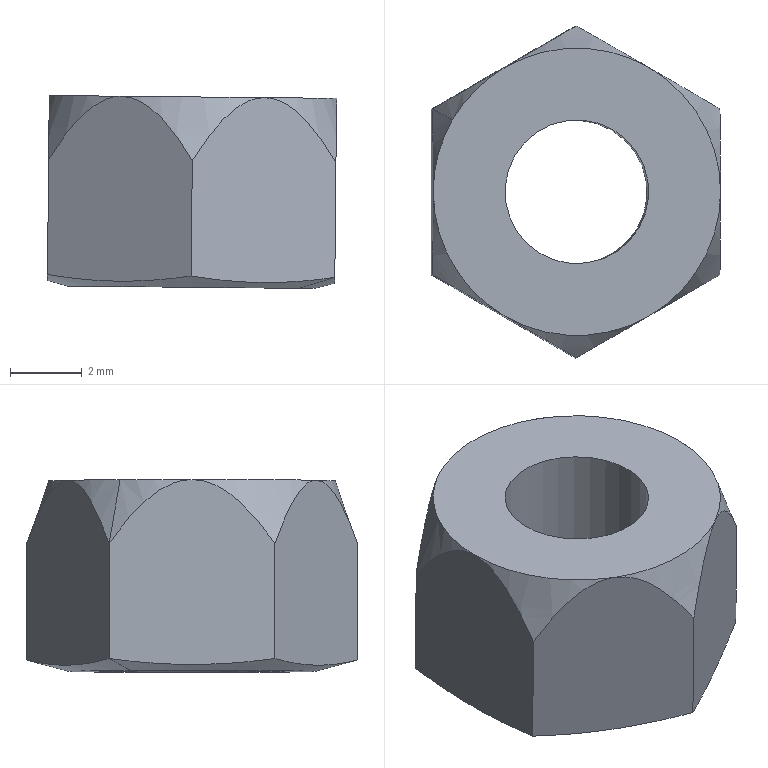Component | SolidWorks | prevailing torque all-metal 1 gb M4-6 | 1 solid | 21 faces | box 8.05 x 9.24 x 5.37 mm | volume 220 mm3 | cone 11 | plane 8 | cylinder 2 | commonest cylinder face diameters 4 x2
STEP:
#1=COLOUR_RGB('',0.7922,0.8196,0.9333);
#2=FILL_AREA_STYLE_COLOUR('',#1);
#3=FILL_AREA_STYLE('',(#2));
#4=SURFACE_STYLE_FILL_AREA(#3);
#5=SURFACE_SIDE_STYLE('',(#4));
#6=SURFACE_STYLE_USAGE(.BOTH.,#5);
#7=PRESENTATION_STYLE_ASSIGNMENT((#6));
#8=CARTESIAN_POINT('',(1.238,0.9643,-0.07411));
#9=VERTEX_POINT('',#8);
#10=CARTESIAN_POINT('',(1.101,1.043,-0.07277));
#11=VERTEX_POINT('',#10);
#12=CARTESIAN_POINT('',(1.169,1.004,-0.07344));
#13=DIRECTION('',(-0.009793,0.,-1.));
#14=DIRECTION('',(-0.866,0.5,0.008481));
#15=AXIS2_PLACEMENT_3D('',#12,#13,#14);
#16=CIRCLE('',#15,0.07874);
#17=EDGE_CURVE('',#9,#11,#16,.T.);
#18=ORIENTED_EDGE('',*,*,#17,.F.);
#19=CARTESIAN_POINT('',(1.257,0.9531,-0.0968));
#20=VERTEX_POINT('',#19);
#21=CARTESIAN_POINT('',(1.257,0.9531,-0.0968));
#22=DIRECTION('',(0.6054,-0.3536,-0.7131));
#23=VECTOR('',#22,39.37);
#24=LINE('',#21,#23);
#25=EDGE_CURVE('',#9,#20,#24,.T.);
#26=ORIENTED_EDGE('',*,*,#25,.T.);
#27=CARTESIAN_POINT('',(1.082,1.054,-0.09508));
#28=VERTEX_POINT('',#27);
#29=CARTESIAN_POINT('',(1.169,1.004,-0.09594));
#30=DIRECTION('',(0.009793,-0.,1.));
#31=DIRECTION('',(-0.866,0.5,0.008481));
#32=AXIS2_PLACEMENT_3D('',#29,#30,#31);
#33=CIRCLE('',#32,0.1012);
#34=EDGE_CURVE('',#28,#20,#33,.T.);
#35=ORIENTED_EDGE('',*,*,#34,.F.);
#36=CARTESIAN_POINT('',(1.082,1.054,-0.09508));
#37=DIRECTION('',(-0.6193,0.3536,-0.7011));
#38=VECTOR('',#37,39.37);
#39=LINE('',#36,#38);
#40=EDGE_CURVE('',#11,#28,#39,.T.);
#41=ORIENTED_EDGE('',*,*,#40,.F.);
#42=EDGE_LOOP('',(#18,#26,#35,#41));
#43=FACE_OUTER_BOUND('',#42,.T.);
#44=CARTESIAN_POINT('',(1.169,1.004,-0.09594));
#45=DIRECTION('',(-0.009793,0.,-1.));
#46=DIRECTION('',(-0.866,0.5,0.008481));
#47=AXIS2_PLACEMENT_3D('',#44,#45,#46);
#48=CONICAL_SURFACE('',#47,0.1012,0.7854);
#49=ADVANCED_FACE('',(#43),#48,.F.);
#50=ORIENTED_EDGE('',*,*,#17,.T.);
#51=CARTESIAN_POINT('',(1.103,1.043,0.1134));
#52=VERTEX_POINT('',#51);
#53=CARTESIAN_POINT('',(1.101,1.043,-0.09527));
#54=DIRECTION('',(0.009793,-0.,1.));
#55=VECTOR('',#54,39.37);
#56=LINE('',#53,#55);
#57=EDGE_CURVE('',#11,#52,#56,.T.);
#58=ORIENTED_EDGE('',*,*,#57,.T.);
#59=CARTESIAN_POINT('',(1.239,0.9643,0.112));
#60=VERTEX_POINT('',#59);
#61=CARTESIAN_POINT('',(1.171,1.004,0.1127));
#62=DIRECTION('',(0.009793,-0.,1.));
#63=DIRECTION('',(0.866,-0.5,-0.008481));
#64=AXIS2_PLACEMENT_3D('',#61,#62,#63);
#65=CIRCLE('',#64,0.07874);
#66=EDGE_CURVE('',#52,#60,#65,.T.);
#67=ORIENTED_EDGE('',*,*,#66,.T.);
#68=CARTESIAN_POINT('',(1.237,0.9643,-0.09661));
#69=DIRECTION('',(0.009793,-0.,1.));
#70=VECTOR('',#69,39.37);
#71=LINE('',#68,#70);
#72=EDGE_CURVE('',#9,#60,#71,.T.);
#73=ORIENTED_EDGE('',*,*,#72,.F.);
#74=EDGE_LOOP('',(#50,#58,#67,#73));
#75=FACE_OUTER_BOUND('',#74,.T.);
#76=CARTESIAN_POINT('',(1.169,1.004,-0.09594));
#77=DIRECTION('',(0.009793,-0.,1.));
#78=DIRECTION('',(0.866,-0.5,-0.008481));
#79=AXIS2_PLACEMENT_3D('',#76,#77,#78);
#80=CYLINDRICAL_SURFACE('',#79,0.07874);
#81=ADVANCED_FACE('',(#75),#80,.F.);
#82=CARTESIAN_POINT('',(1.035,1.082,0.114));
#83=VERTEX_POINT('',#82);
#84=CARTESIAN_POINT('',(1.014,1.004,0.1143));
#85=VERTEX_POINT('',#84);
#86=CARTESIAN_POINT('',(1.171,1.004,0.1127));
#87=DIRECTION('',(0.009793,-0.,1.));
#88=DIRECTION('',(-0.866,0.5,0.008481));
#89=AXIS2_PLACEMENT_3D('',#86,#87,#88);
#90=CIRCLE('',#89,0.1575);
#91=EDGE_CURVE('',#83,#85,#90,.T.);
#92=ORIENTED_EDGE('',*,*,#91,.F.);
#93=CARTESIAN_POINT('',(1.013,1.095,0.04418));
#94=VERTEX_POINT('',#93);
#95=CARTESIAN_POINT('',(1.035,1.082,0.114));
#96=DIRECTION('',(-0.2936,0.1642,-0.9417));
#97=VECTOR('',#96,39.37);
#98=LINE('',#95,#97);
#99=EDGE_CURVE('',#83,#94,#98,.T.);
#100=ORIENTED_EDGE('',*,*,#99,.T.);
#101=CARTESIAN_POINT('',(1.013,1.095,0.04418));
#102=CARTESIAN_POINT('',(1.013,1.089,0.05232));
#103=CARTESIAN_POINT('',(1.013,1.083,0.06026));
#104=CARTESIAN_POINT('',(1.013,1.07,0.07546));
#105=CARTESIAN_POINT('',(1.013,1.064,0.08273));
#106=CARTESIAN_POINT('',(1.014,1.049,0.09611));
#107=CARTESIAN_POINT('',(1.014,1.041,0.1022));
#108=CARTESIAN_POINT('',(1.014,1.024,0.1114));
#109=CARTESIAN_POINT('',(1.014,1.014,0.1143));
#110=CARTESIAN_POINT('',(1.014,1.004,0.1143));
#111=B_SPLINE_CURVE_WITH_KNOTS('',3,(#101,#102,#103,#104,#105,#106,#107,#108,#109,#110),.UNSPECIFIED.,.F.,.F.,(4,2,2,2,4),(0.00000024,0.000751,0.001502,0.002252,0.003003),.UNSPECIFIED.);
#112=EDGE_CURVE('',#94,#85,#111,.T.);
#113=ORIENTED_EDGE('',*,*,#112,.T.);
#114=EDGE_LOOP('',(#92,#100,#113));
#115=FACE_OUTER_BOUND('',#114,.T.);
#116=CARTESIAN_POINT('',(1.171,1.004,0.1127));
#117=DIRECTION('',(-0.009793,0.,-1.));
#118=DIRECTION('',(-0.866,0.5,0.008481));
#119=AXIS2_PLACEMENT_3D('',#116,#117,#118);
#120=CONICAL_SURFACE('',#119,0.1575,0.3346);
#121=ADVANCED_FACE('',(#115),#120,.T.);
#122=CARTESIAN_POINT('',(1.052,1.071,-0.09479));
#123=VERTEX_POINT('',#122);
#124=CARTESIAN_POINT('',(1.286,0.936,-0.09709));
#125=VERTEX_POINT('',#124);
#126=CARTESIAN_POINT('',(1.169,1.004,-0.09594));
#127=DIRECTION('',(-0.009793,0.,-1.));
#128=DIRECTION('',(-0.866,0.5,0.008481));
#129=AXIS2_PLACEMENT_3D('',#126,#127,#128);
#130=CIRCLE('',#129,0.1354);
#131=EDGE_CURVE('',#123,#125,#130,.T.);
#132=ORIENTED_EDGE('',*,*,#131,.F.);
#133=CARTESIAN_POINT('',(1.012,1.095,-0.08196));
#134=VERTEX_POINT('',#133);
#135=CARTESIAN_POINT('',(1.012,1.095,-0.08196));
#136=DIRECTION('',(-0.8339,0.483,0.267));
#137=VECTOR('',#136,39.37);
#138=LINE('',#135,#137);
#139=EDGE_CURVE('',#123,#134,#138,.T.);
#140=ORIENTED_EDGE('',*,*,#139,.T.);
#141=CARTESIAN_POINT('',(1.169,1.186,-0.0835));
#142=VERTEX_POINT('',#141);
#143=CARTESIAN_POINT('',(1.012,1.095,-0.08196));
#144=CARTESIAN_POINT('',(1.038,1.11,-0.08628));
#145=CARTESIAN_POINT('',(1.091,1.14,-0.09173));
#146=CARTESIAN_POINT('',(1.143,1.17,-0.08731));
#147=CARTESIAN_POINT('',(1.169,1.186,-0.0835));
#148=B_SPLINE_CURVE_WITH_KNOTS('',3,(#143,#144,#145,#146,#147),.UNSPECIFIED.,.F.,.F.,(4,1,4),(0.00000023,0.00231,0.004619),.UNSPECIFIED.);
#149=EDGE_CURVE('',#134,#142,#148,.T.);
#150=ORIENTED_EDGE('',*,*,#149,.T.);
#151=CARTESIAN_POINT('',(1.327,1.095,-0.08505));
#152=VERTEX_POINT('',#151);
#153=CARTESIAN_POINT('',(1.169,1.186,-0.0835));
#154=CARTESIAN_POINT('',(1.182,1.178,-0.08566));
#155=CARTESIAN_POINT('',(1.196,1.17,-0.08745));
#156=CARTESIAN_POINT('',(1.222,1.155,-0.08996));
#157=CARTESIAN_POINT('',(1.235,1.148,-0.09068));
#158=CARTESIAN_POINT('',(1.274,1.125,-0.09105));
#159=CARTESIAN_POINT('',(1.301,1.11,-0.08883));
#160=CARTESIAN_POINT('',(1.327,1.095,-0.08505));
#161=B_SPLINE_CURVE_WITH_KNOTS('',3,(#153,#154,#155,#156,#157,#158,#159,#160),.UNSPECIFIED.,.F.,.F.,(4,2,2,4),(0.003852,0.005015,0.006177,0.008501),.UNSPECIFIED.);
#162=EDGE_CURVE('',#142,#152,#161,.T.);
#163=ORIENTED_EDGE('',*,*,#162,.T.);
#164=CARTESIAN_POINT('',(1.327,0.9128,-0.08505));
#165=VERTEX_POINT('',#164);
#166=CARTESIAN_POINT('',(1.327,1.095,-0.08505));
#167=CARTESIAN_POINT('',(1.327,1.064,-0.08911));
#168=CARTESIAN_POINT('',(1.327,1.004,-0.09404));
#169=CARTESIAN_POINT('',(1.327,0.9431,-0.08911));
#170=CARTESIAN_POINT('',(1.327,0.9128,-0.08505));
#171=B_SPLINE_CURVE_WITH_KNOTS('',3,(#166,#167,#168,#169,#170),.UNSPECIFIED.,.F.,.F.,(4,1,4),(0.00000023,0.00231,0.004619),.UNSPECIFIED.);
#172=EDGE_CURVE('',#152,#165,#171,.T.);
#173=ORIENTED_EDGE('',*,*,#172,.T.);
#174=CARTESIAN_POINT('',(1.327,0.9128,-0.08505));
#175=DIRECTION('',(0.839,-0.483,0.2506));
#176=VECTOR('',#175,39.37);
#177=LINE('',#174,#176);
#178=EDGE_CURVE('',#125,#165,#177,.T.);
#179=ORIENTED_EDGE('',*,*,#178,.F.);
#180=EDGE_LOOP('',(#132,#140,#150,#163,#173,#179));
#181=FACE_OUTER_BOUND('',#180,.T.);
#182=CARTESIAN_POINT('',(1.169,1.004,-0.0835));
#183=DIRECTION('',(0.009793,-0.,1.));
#184=DIRECTION('',(0.866,-0.5,-0.008481));
#185=AXIS2_PLACEMENT_3D('',#182,#183,#184);
#186=CONICAL_SURFACE('',#185,0.1818,1.309);
#187=ADVANCED_FACE('',(#181),#186,.T.);
#188=CARTESIAN_POINT('',(1.013,0.9128,0.04418));
#189=VERTEX_POINT('',#188);
#190=CARTESIAN_POINT('',(1.093,0.8673,0.1135));
#191=VERTEX_POINT('',#190);
#192=CARTESIAN_POINT('',(1.013,0.9128,0.04418));
#193=CARTESIAN_POINT('',(1.018,0.91,0.05219));
#194=CARTESIAN_POINT('',(1.023,0.907,0.06004));
#195=CARTESIAN_POINT('',(1.034,0.9007,0.0752));
#196=CARTESIAN_POINT('',(1.04,0.8973,0.08254));
#197=CARTESIAN_POINT('',(1.053,0.89,0.0958));
#198=CARTESIAN_POINT('',(1.06,0.886,0.1019));
#199=CARTESIAN_POINT('',(1.071,0.8794,0.1085));
#200=CARTESIAN_POINT('',(1.076,0.8771,0.1104));
#201=CARTESIAN_POINT('',(1.084,0.8723,0.1129));
#202=CARTESIAN_POINT('',(1.088,0.8698,0.1135));
#203=CARTESIAN_POINT('',(1.093,0.8673,0.1135));
#204=B_SPLINE_CURVE_WITH_KNOTS('',3,(#192,#193,#194,#195,#196,#197,#198,#199,#200,#201,#202,#203),.UNSPECIFIED.,.F.,.F.,(4,2,2,2,2,4),(0.003325,0.004072,0.004819,0.005566,0.00594,0.006313),.UNSPECIFIED.);
#205=EDGE_CURVE('',#189,#191,#204,.T.);
#206=ORIENTED_EDGE('',*,*,#205,.F.);
#207=CARTESIAN_POINT('',(1.012,0.9128,-0.08196));
#208=VERTEX_POINT('',#207);
#209=CARTESIAN_POINT('',(1.012,0.9128,-0.0944));
#210=DIRECTION('',(0.009793,-0.,1.));
#211=VECTOR('',#210,39.37);
#212=LINE('',#209,#211);
#213=EDGE_CURVE('',#208,#189,#212,.T.);
#214=ORIENTED_EDGE('',*,*,#213,.F.);
#215=CARTESIAN_POINT('',(1.169,0.8218,-0.0835));
#216=VERTEX_POINT('',#215);
#217=CARTESIAN_POINT('',(1.169,0.8218,-0.0835));
#218=CARTESIAN_POINT('',(1.143,0.8369,-0.08729));
#219=CARTESIAN_POINT('',(1.117,0.8521,-0.08951));
#220=CARTESIAN_POINT('',(1.078,0.8748,-0.08914));
#221=CARTESIAN_POINT('',(1.064,0.8824,-0.08841));
#222=CARTESIAN_POINT('',(1.038,0.8976,-0.0859));
#223=CARTESIAN_POINT('',(1.025,0.9052,-0.08412));
#224=CARTESIAN_POINT('',(1.012,0.9128,-0.08196));
#225=B_SPLINE_CURVE_WITH_KNOTS('',3,(#217,#218,#219,#220,#221,#222,#223,#224),.UNSPECIFIED.,.F.,.F.,(4,2,2,4),(0.008829,0.01115,0.01231,0.01347),.UNSPECIFIED.);
#226=EDGE_CURVE('',#216,#208,#225,.T.);
#227=ORIENTED_EDGE('',*,*,#226,.F.);
#228=CARTESIAN_POINT('',(1.171,0.8218,0.04264));
#229=VERTEX_POINT('',#228);
#230=CARTESIAN_POINT('',(1.169,0.8218,-0.09594));
#231=DIRECTION('',(0.009793,-0.,1.));
#232=VECTOR('',#231,39.37);
#233=LINE('',#230,#232);
#234=EDGE_CURVE('',#216,#229,#233,.T.);
#235=ORIENTED_EDGE('',*,*,#234,.T.);
#236=CARTESIAN_POINT('',(1.093,0.8673,0.1135));
#237=CARTESIAN_POINT('',(1.101,0.8623,0.1134));
#238=CARTESIAN_POINT('',(1.11,0.8573,0.1104));
#239=CARTESIAN_POINT('',(1.125,0.8485,0.1011));
#240=CARTESIAN_POINT('',(1.132,0.8445,0.09493));
#241=CARTESIAN_POINT('',(1.144,0.8372,0.08143));
#242=CARTESIAN_POINT('',(1.15,0.8339,0.0741));
#243=CARTESIAN_POINT('',(1.161,0.8276,0.0588));
#244=CARTESIAN_POINT('',(1.166,0.8247,0.05082));
#245=CARTESIAN_POINT('',(1.171,0.8218,0.04264));
#246=B_SPLINE_CURVE_WITH_KNOTS('',3,(#236,#237,#238,#239,#240,#241,#242,#243,#244,#245),.UNSPECIFIED.,.F.,.F.,(4,2,2,2,4),(0.006313,0.007062,0.007811,0.00856,0.009309),.UNSPECIFIED.);
#247=EDGE_CURVE('',#191,#229,#246,.T.);
#248=ORIENTED_EDGE('',*,*,#247,.F.);
#249=EDGE_LOOP('',(#206,#214,#227,#235,#248));
#250=FACE_OUTER_BOUND('',#249,.T.);
#251=CARTESIAN_POINT('',(1.012,0.9128,-0.0944));
#252=DIRECTION('',(-0.5,-0.866,0.004897));
#253=DIRECTION('',(-0.009793,0.,-1.));
#254=AXIS2_PLACEMENT_3D('',#251,#252,#253);
#255=PLANE('',#254);
#256=ADVANCED_FACE('',(#250),#255,.T.);
#257=ORIENTED_EDGE('',*,*,#112,.F.);
#258=CARTESIAN_POINT('',(1.012,1.095,-0.0944));
#259=DIRECTION('',(0.009793,-0.,1.));
#260=VECTOR('',#259,39.37);
#261=LINE('',#258,#260);
#262=EDGE_CURVE('',#134,#94,#261,.T.);
#263=ORIENTED_EDGE('',*,*,#262,.F.);
#264=CARTESIAN_POINT('',(1.012,0.9128,-0.08196));
#265=CARTESIAN_POINT('',(1.012,0.9431,-0.08602));
#266=CARTESIAN_POINT('',(1.012,1.004,-0.09096));
#267=CARTESIAN_POINT('',(1.012,1.064,-0.08602));
#268=CARTESIAN_POINT('',(1.012,1.095,-0.08196));
#269=B_SPLINE_CURVE_WITH_KNOTS('',3,(#264,#265,#266,#267,#268),.UNSPECIFIED.,.F.,.F.,(4,1,4),(0.00000023,0.00231,0.004619),.UNSPECIFIED.);
#270=EDGE_CURVE('',#208,#134,#269,.T.);
#271=ORIENTED_EDGE('',*,*,#270,.F.);
#272=ORIENTED_EDGE('',*,*,#213,.T.);
#273=CARTESIAN_POINT('',(1.014,1.004,0.1143));
#274=CARTESIAN_POINT('',(1.014,0.9937,0.1143));
#275=CARTESIAN_POINT('',(1.014,0.9839,0.1114));
#276=CARTESIAN_POINT('',(1.014,0.9663,0.1023));
#277=CARTESIAN_POINT('',(1.014,0.9583,0.09621));
#278=CARTESIAN_POINT('',(1.013,0.9437,0.0829));
#279=CARTESIAN_POINT('',(1.013,0.937,0.07561));
#280=CARTESIAN_POINT('',(1.013,0.9244,0.06031));
#281=CARTESIAN_POINT('',(1.013,0.9184,0.05233));
#282=CARTESIAN_POINT('',(1.013,0.9128,0.04418));
#283=B_SPLINE_CURVE_WITH_KNOTS('',3,(#273,#274,#275,#276,#277,#278,#279,#280,#281,#282),.UNSPECIFIED.,.F.,.F.,(4,2,2,2,4),(0.003003,0.003753,0.004503,0.005252,0.006002),.UNSPECIFIED.);
#284=EDGE_CURVE('',#85,#189,#283,.T.);
#285=ORIENTED_EDGE('',*,*,#284,.F.);
#286=EDGE_LOOP('',(#257,#263,#271,#272,#285));
#287=FACE_OUTER_BOUND('',#286,.T.);
#288=CARTESIAN_POINT('',(1.012,1.095,-0.0944));
#289=DIRECTION('',(-1.,0.,0.009793));
#290=DIRECTION('',(-0.,-1.,-0.));
#291=AXIS2_PLACEMENT_3D('',#288,#289,#290);
#292=PLANE('',#291);
#293=ADVANCED_FACE('',(#287),#292,.T.);
#294=CARTESIAN_POINT('',(1.171,1.186,0.04264));
#295=VERTEX_POINT('',#294);
#296=CARTESIAN_POINT('',(1.093,1.14,0.1135));
#297=VERTEX_POINT('',#296);
#298=CARTESIAN_POINT('',(1.171,1.186,0.04264));
#299=CARTESIAN_POINT('',(1.166,1.183,0.05083));
#300=CARTESIAN_POINT('',(1.161,1.18,0.05881));
#301=CARTESIAN_POINT('',(1.15,1.173,0.07412));
#302=CARTESIAN_POINT('',(1.144,1.17,0.08145));
#303=CARTESIAN_POINT('',(1.132,1.163,0.09496));
#304=CARTESIAN_POINT('',(1.125,1.159,0.1011));
#305=CARTESIAN_POINT('',(1.11,1.15,0.1104));
#306=CARTESIAN_POINT('',(1.101,1.145,0.1134));
#307=CARTESIAN_POINT('',(1.093,1.14,0.1135));
#308=B_SPLINE_CURVE_WITH_KNOTS('',3,(#298,#299,#300,#301,#302,#303,#304,#305,#306,#307),.UNSPECIFIED.,.F.,.F.,(4,2,2,2,4),(0.00000024,0.000751,0.001502,0.002252,0.003003),.UNSPECIFIED.);
#309=EDGE_CURVE('',#295,#297,#308,.T.);
#310=ORIENTED_EDGE('',*,*,#309,.F.);
#311=CARTESIAN_POINT('',(1.169,1.186,-0.09594));
#312=DIRECTION('',(0.009793,-0.,1.));
#313=VECTOR('',#312,39.37);
#314=LINE('',#311,#313);
#315=EDGE_CURVE('',#142,#295,#314,.T.);
#316=ORIENTED_EDGE('',*,*,#315,.F.);
#317=ORIENTED_EDGE('',*,*,#149,.F.);
#318=ORIENTED_EDGE('',*,*,#262,.T.);
#319=CARTESIAN_POINT('',(1.093,1.14,0.1135));
#320=CARTESIAN_POINT('',(1.084,1.135,0.1136));
#321=CARTESIAN_POINT('',(1.075,1.13,0.1108));
#322=CARTESIAN_POINT('',(1.06,1.121,0.1019));
#323=CARTESIAN_POINT('',(1.053,1.117,0.09583));
#324=CARTESIAN_POINT('',(1.04,1.11,0.08264));
#325=CARTESIAN_POINT('',(1.034,1.107,0.0754));
#326=CARTESIAN_POINT('',(1.023,1.1,0.06021));
#327=CARTESIAN_POINT('',(1.018,1.097,0.05229));
#328=CARTESIAN_POINT('',(1.013,1.095,0.04418));
#329=B_SPLINE_CURVE_WITH_KNOTS('',3,(#319,#320,#321,#322,#323,#324,#325,#326,#327,#328),.UNSPECIFIED.,.F.,.F.,(4,2,2,2,4),(0.003003,0.003753,0.004503,0.005252,0.006002),.UNSPECIFIED.);
#330=EDGE_CURVE('',#297,#94,#329,.T.);
#331=ORIENTED_EDGE('',*,*,#330,.F.);
#332=EDGE_LOOP('',(#310,#316,#317,#318,#331));
#333=FACE_OUTER_BOUND('',#332,.T.);
#334=CARTESIAN_POINT('',(1.169,1.186,-0.09594));
#335=DIRECTION('',(-0.5,0.866,0.004897));
#336=DIRECTION('',(-0.866,-0.5,0.008481));
#337=AXIS2_PLACEMENT_3D('',#334,#335,#336);
#338=PLANE('',#337);
#339=ADVANCED_FACE('',(#333),#338,.T.);
#340=CARTESIAN_POINT('',(1.328,1.095,0.0411));
#341=VERTEX_POINT('',#340);
#342=CARTESIAN_POINT('',(1.25,1.14,0.1119));
#343=VERTEX_POINT('',#342);
#344=CARTESIAN_POINT('',(1.328,1.095,0.0411));
#345=CARTESIAN_POINT('',(1.323,1.097,0.04928));
#346=CARTESIAN_POINT('',(1.318,1.1,0.05726));
#347=CARTESIAN_POINT('',(1.307,1.107,0.07256));
#348=CARTESIAN_POINT('',(1.302,1.11,0.07989));
#349=CARTESIAN_POINT('',(1.289,1.117,0.09339));
#350=CARTESIAN_POINT('',(1.282,1.121,0.0996));
#351=CARTESIAN_POINT('',(1.267,1.13,0.1089));
#352=CARTESIAN_POINT('',(1.259,1.135,0.1119));
#353=CARTESIAN_POINT('',(1.25,1.14,0.1119));
#354=B_SPLINE_CURVE_WITH_KNOTS('',3,(#344,#345,#346,#347,#348,#349,#350,#351,#352,#353),.UNSPECIFIED.,.F.,.F.,(4,2,2,2,4),(0.008014,0.008762,0.00951,0.01026,0.01101),.UNSPECIFIED.);
#355=EDGE_CURVE('',#341,#343,#354,.T.);
#356=ORIENTED_EDGE('',*,*,#355,.F.);
#357=CARTESIAN_POINT('',(1.327,1.095,-0.09748));
#358=DIRECTION('',(0.009793,-0.,1.));
#359=VECTOR('',#358,39.37);
#360=LINE('',#357,#359);
#361=EDGE_CURVE('',#152,#341,#360,.T.);
#362=ORIENTED_EDGE('',*,*,#361,.F.);
#363=ORIENTED_EDGE('',*,*,#162,.F.);
#364=ORIENTED_EDGE('',*,*,#315,.T.);
#365=CARTESIAN_POINT('',(1.25,1.14,0.1119));
#366=CARTESIAN_POINT('',(1.246,1.143,0.112));
#367=CARTESIAN_POINT('',(1.241,1.145,0.1113));
#368=CARTESIAN_POINT('',(1.233,1.15,0.1088));
#369=CARTESIAN_POINT('',(1.229,1.152,0.107));
#370=CARTESIAN_POINT('',(1.217,1.159,0.1003));
#371=CARTESIAN_POINT('',(1.21,1.163,0.09426));
#372=CARTESIAN_POINT('',(1.198,1.17,0.081));
#373=CARTESIAN_POINT('',(1.192,1.173,0.07365));
#374=CARTESIAN_POINT('',(1.181,1.18,0.0585));
#375=CARTESIAN_POINT('',(1.175,1.183,0.05065));
#376=CARTESIAN_POINT('',(1.171,1.186,0.04264));
#377=B_SPLINE_CURVE_WITH_KNOTS('',3,(#365,#366,#367,#368,#369,#370,#371,#372,#373,#374,#375,#376),.UNSPECIFIED.,.F.,.F.,(4,2,2,2,2,4),(0.01101,0.01138,0.01175,0.0125,0.01324,0.01399),.UNSPECIFIED.);
#378=EDGE_CURVE('',#343,#295,#377,.T.);
#379=ORIENTED_EDGE('',*,*,#378,.F.);
#380=EDGE_LOOP('',(#356,#362,#363,#364,#379));
#381=FACE_OUTER_BOUND('',#380,.T.);
#382=CARTESIAN_POINT('',(1.327,1.095,-0.09748));
#383=DIRECTION('',(0.5,0.866,-0.004897));
#384=DIRECTION('',(0.009793,-0.,1.));
#385=AXIS2_PLACEMENT_3D('',#382,#383,#384);
#386=PLANE('',#385);
#387=ADVANCED_FACE('',(#381),#386,.T.);
#388=CARTESIAN_POINT('',(1.328,0.9128,0.0411));
#389=VERTEX_POINT('',#388);
#390=CARTESIAN_POINT('',(1.329,1.004,0.1112));
#391=VERTEX_POINT('',#390);
#392=CARTESIAN_POINT('',(1.328,0.9128,0.0411));
#393=CARTESIAN_POINT('',(1.328,0.9184,0.04924));
#394=CARTESIAN_POINT('',(1.328,0.9243,0.05717));
#395=CARTESIAN_POINT('',(1.328,0.9369,0.07237));
#396=CARTESIAN_POINT('',(1.328,0.9435,0.07965));
#397=CARTESIAN_POINT('',(1.329,0.9581,0.09303));
#398=CARTESIAN_POINT('',(1.329,0.9661,0.09915));
#399=CARTESIAN_POINT('',(1.329,0.9838,0.1083));
#400=CARTESIAN_POINT('',(1.329,0.9937,0.1112));
#401=CARTESIAN_POINT('',(1.329,1.004,0.1112));
#402=B_SPLINE_CURVE_WITH_KNOTS('',3,(#392,#393,#394,#395,#396,#397,#398,#399,#400,#401),.UNSPECIFIED.,.F.,.F.,(4,2,2,2,4),(0.00000024,0.000751,0.001502,0.002252,0.003003),.UNSPECIFIED.);
#403=EDGE_CURVE('',#389,#391,#402,.T.);
#404=ORIENTED_EDGE('',*,*,#403,.F.);
#405=CARTESIAN_POINT('',(1.327,0.9128,-0.09748));
#406=DIRECTION('',(0.009793,-0.,1.));
#407=VECTOR('',#406,39.37);
#408=LINE('',#405,#407);
#409=EDGE_CURVE('',#165,#389,#408,.T.);
#410=ORIENTED_EDGE('',*,*,#409,.F.);
#411=ORIENTED_EDGE('',*,*,#172,.F.);
#412=ORIENTED_EDGE('',*,*,#361,.T.);
#413=CARTESIAN_POINT('',(1.329,1.004,0.1112));
#414=CARTESIAN_POINT('',(1.329,1.014,0.1112));
#415=CARTESIAN_POINT('',(1.329,1.023,0.1083));
#416=CARTESIAN_POINT('',(1.329,1.041,0.09925));
#417=CARTESIAN_POINT('',(1.329,1.049,0.09313));
#418=CARTESIAN_POINT('',(1.328,1.064,0.07982));
#419=CARTESIAN_POINT('',(1.328,1.07,0.07252));
#420=CARTESIAN_POINT('',(1.328,1.083,0.05722));
#421=CARTESIAN_POINT('',(1.328,1.089,0.04925));
#422=CARTESIAN_POINT('',(1.328,1.095,0.0411));
#423=B_SPLINE_CURVE_WITH_KNOTS('',3,(#413,#414,#415,#416,#417,#418,#419,#420,#421,#422),.UNSPECIFIED.,.F.,.F.,(4,2,2,2,4),(0.003003,0.003753,0.004503,0.005252,0.006002),.UNSPECIFIED.);
#424=EDGE_CURVE('',#391,#341,#423,.T.);
#425=ORIENTED_EDGE('',*,*,#424,.F.);
#426=EDGE_LOOP('',(#404,#410,#411,#412,#425));
#427=FACE_OUTER_BOUND('',#426,.T.);
#428=CARTESIAN_POINT('',(1.327,0.9128,-0.09748));
#429=DIRECTION('',(1.,-0.,-0.009793));
#430=DIRECTION('',(0.,1.,0.));
#431=AXIS2_PLACEMENT_3D('',#428,#429,#430);
#432=PLANE('',#431);
#433=ADVANCED_FACE('',(#427),#432,.T.);
#434=CARTESIAN_POINT('',(1.25,0.8673,0.1119));
#435=VERTEX_POINT('',#434);
#436=CARTESIAN_POINT('',(1.171,0.8218,0.04264));
#437=CARTESIAN_POINT('',(1.176,0.8247,0.05073));
#438=CARTESIAN_POINT('',(1.181,0.8276,0.05861));
#439=CARTESIAN_POINT('',(1.192,0.8339,0.07371));
#440=CARTESIAN_POINT('',(1.198,0.8372,0.08093));
#441=CARTESIAN_POINT('',(1.21,0.8445,0.09419));
#442=CARTESIAN_POINT('',(1.217,0.8485,0.1002));
#443=CARTESIAN_POINT('',(1.233,0.8574,0.1092));
#444=CARTESIAN_POINT('',(1.241,0.8623,0.112));
#445=CARTESIAN_POINT('',(1.25,0.8673,0.1119));
#446=B_SPLINE_CURVE_WITH_KNOTS('',3,(#436,#437,#438,#439,#440,#441,#442,#443,#444,#445),.UNSPECIFIED.,.F.,.F.,(4,2,2,2,4),(0.00000024,0.000751,0.001502,0.002252,0.003003),.UNSPECIFIED.);
#447=EDGE_CURVE('',#229,#435,#446,.T.);
#448=ORIENTED_EDGE('',*,*,#447,.F.);
#449=ORIENTED_EDGE('',*,*,#234,.F.);
#450=CARTESIAN_POINT('',(1.327,0.9128,-0.08505));
#451=CARTESIAN_POINT('',(1.301,0.8976,-0.08885));
#452=CARTESIAN_POINT('',(1.248,0.8673,-0.09327));
#453=CARTESIAN_POINT('',(1.196,0.837,-0.08782));
#454=CARTESIAN_POINT('',(1.169,0.8218,-0.0835));
#455=B_SPLINE_CURVE_WITH_KNOTS('',3,(#450,#451,#452,#453,#454),.UNSPECIFIED.,.F.,.F.,(4,1,4),(0.00000023,0.00231,0.004619),.UNSPECIFIED.);
#456=EDGE_CURVE('',#165,#216,#455,.T.);
#457=ORIENTED_EDGE('',*,*,#456,.F.);
#458=ORIENTED_EDGE('',*,*,#409,.T.);
#459=CARTESIAN_POINT('',(1.25,0.8673,0.1119));
#460=CARTESIAN_POINT('',(1.259,0.8723,0.1119));
#461=CARTESIAN_POINT('',(1.267,0.8772,0.1089));
#462=CARTESIAN_POINT('',(1.282,0.886,0.0997));
#463=CARTESIAN_POINT('',(1.289,0.89,0.09351));
#464=CARTESIAN_POINT('',(1.302,0.8973,0.08008));
#465=CARTESIAN_POINT('',(1.307,0.9006,0.07273));
#466=CARTESIAN_POINT('',(1.318,0.907,0.05732));
#467=CARTESIAN_POINT('',(1.323,0.9099,0.0493));
#468=CARTESIAN_POINT('',(1.328,0.9128,0.0411));
#469=B_SPLINE_CURVE_WITH_KNOTS('',3,(#459,#460,#461,#462,#463,#464,#465,#466,#467,#468),.UNSPECIFIED.,.F.,.F.,(4,2,2,2,4),(0.003003,0.003753,0.004503,0.005252,0.006002),.UNSPECIFIED.);
#470=EDGE_CURVE('',#435,#389,#469,.T.);
#471=ORIENTED_EDGE('',*,*,#470,.F.);
#472=EDGE_LOOP('',(#448,#449,#457,#458,#471));
#473=FACE_OUTER_BOUND('',#472,.T.);
#474=CARTESIAN_POINT('',(1.169,0.8218,-0.09594));
#475=DIRECTION('',(0.5,-0.866,-0.004897));
#476=DIRECTION('',(0.866,0.5,-0.008481));
#477=AXIS2_PLACEMENT_3D('',#474,#475,#476);
#478=PLANE('',#477);
#479=ADVANCED_FACE('',(#473),#478,.T.);
#480=ORIENTED_EDGE('',*,*,#139,.F.);
#481=CARTESIAN_POINT('',(1.169,1.004,-0.09594));
#482=DIRECTION('',(-0.009793,0.,-1.));
#483=DIRECTION('',(-0.866,0.5,0.008481));
#484=AXIS2_PLACEMENT_3D('',#481,#482,#483);
#485=CIRCLE('',#484,0.1354);
#486=EDGE_CURVE('',#125,#123,#485,.T.);
#487=ORIENTED_EDGE('',*,*,#486,.F.);
#488=ORIENTED_EDGE('',*,*,#178,.T.);
#489=ORIENTED_EDGE('',*,*,#456,.T.);
#490=ORIENTED_EDGE('',*,*,#226,.T.);
#491=ORIENTED_EDGE('',*,*,#270,.T.);
#492=EDGE_LOOP('',(#480,#487,#488,#489,#490,#491));
#493=FACE_OUTER_BOUND('',#492,.T.);
#494=CARTESIAN_POINT('',(1.169,1.004,-0.0835));
#495=DIRECTION('',(0.009793,-0.,1.));
#496=DIRECTION('',(0.866,-0.5,-0.008481));
#497=AXIS2_PLACEMENT_3D('',#494,#495,#496);
#498=CONICAL_SURFACE('',#497,0.1818,1.309);
#499=ADVANCED_FACE('',(#493),#498,.T.);
#500=ORIENTED_EDGE('',*,*,#34,.T.);
#501=CARTESIAN_POINT('',(1.169,1.004,-0.09594));
#502=DIRECTION('',(0.009793,-0.,1.));
#503=DIRECTION('',(-0.866,0.5,0.008481));
#504=AXIS2_PLACEMENT_3D('',#501,#502,#503);
#505=CIRCLE('',#504,0.1012);
#506=EDGE_CURVE('',#20,#28,#505,.T.);
#507=ORIENTED_EDGE('',*,*,#506,.T.);
#508=EDGE_LOOP('',(#500,#507));
#509=FACE_BOUND('',#508,.T.);
#510=ORIENTED_EDGE('',*,*,#486,.T.);
#511=ORIENTED_EDGE('',*,*,#131,.T.);
#512=EDGE_LOOP('',(#510,#511));
#513=FACE_OUTER_BOUND('',#512,.T.);
#514=CARTESIAN_POINT('',(1.012,0.9128,-0.0944));
#515=DIRECTION('',(-0.009793,0.,-1.));
#516=DIRECTION('',(-0.866,0.5,0.008481));
#517=AXIS2_PLACEMENT_3D('',#514,#515,#516);
#518=PLANE('',#517);
#519=ADVANCED_FACE('',(#509,#513),#518,.T.);
#520=ORIENTED_EDGE('',*,*,#99,.F.);
#521=CARTESIAN_POINT('',(1.171,1.004,0.1127));
#522=DIRECTION('',(0.009793,-0.,1.));
#523=DIRECTION('',(-0.866,0.5,0.008481));
#524=AXIS2_PLACEMENT_3D('',#521,#522,#523);
#525=CIRCLE('',#524,0.1575);
#526=EDGE_CURVE('',#297,#83,#525,.T.);
#527=ORIENTED_EDGE('',*,*,#526,.F.);
#528=ORIENTED_EDGE('',*,*,#330,.T.);
#529=EDGE_LOOP('',(#520,#527,#528));
#530=FACE_OUTER_BOUND('',#529,.T.);
#531=CARTESIAN_POINT('',(1.171,1.004,0.1127));
#532=DIRECTION('',(-0.009793,0.,-1.));
#533=DIRECTION('',(-0.866,0.5,0.008481));
#534=AXIS2_PLACEMENT_3D('',#531,#532,#533);
#535=CONICAL_SURFACE('',#534,0.1575,0.3346);
#536=ADVANCED_FACE('',(#530),#535,.T.);
#537=ORIENTED_EDGE('',*,*,#309,.T.);
#538=CARTESIAN_POINT('',(1.171,1.004,0.1127));
#539=DIRECTION('',(-0.009793,0.,-1.));
#540=DIRECTION('',(-0.866,0.5,0.008481));
#541=AXIS2_PLACEMENT_3D('',#538,#539,#540);
#542=CIRCLE('',#541,0.1575);
#543=EDGE_CURVE('',#297,#343,#542,.T.);
#544=ORIENTED_EDGE('',*,*,#543,.T.);
#545=ORIENTED_EDGE('',*,*,#378,.T.);
#546=EDGE_LOOP('',(#537,#544,#545));
#547=FACE_OUTER_BOUND('',#546,.T.);
#548=CARTESIAN_POINT('',(1.171,1.004,0.1127));
#549=DIRECTION('',(-0.009793,0.,-1.));
#550=DIRECTION('',(-0.866,0.5,0.008481));
#551=AXIS2_PLACEMENT_3D('',#548,#549,#550);
#552=CONICAL_SURFACE('',#551,0.1575,0.3346);
#553=ADVANCED_FACE('',(#547),#552,.T.);
#554=ORIENTED_EDGE('',*,*,#355,.T.);
#555=CARTESIAN_POINT('',(1.171,1.004,0.1127));
#556=DIRECTION('',(0.009793,-0.,1.));
#557=DIRECTION('',(-0.866,0.5,0.008481));
#558=AXIS2_PLACEMENT_3D('',#555,#556,#557);
#559=CIRCLE('',#558,0.1575);
#560=EDGE_CURVE('',#391,#343,#559,.T.);
#561=ORIENTED_EDGE('',*,*,#560,.F.);
#562=ORIENTED_EDGE('',*,*,#424,.T.);
#563=EDGE_LOOP('',(#554,#561,#562));
#564=FACE_OUTER_BOUND('',#563,.T.);
#565=CARTESIAN_POINT('',(1.171,1.004,0.1127));
#566=DIRECTION('',(-0.009793,0.,-1.));
#567=DIRECTION('',(-0.866,0.5,0.008481));
#568=AXIS2_PLACEMENT_3D('',#565,#566,#567);
#569=CONICAL_SURFACE('',#568,0.1575,0.3346);
#570=ADVANCED_FACE('',(#564),#569,.T.);
#571=ORIENTED_EDGE('',*,*,#403,.T.);
#572=CARTESIAN_POINT('',(1.171,1.004,0.1127));
#573=DIRECTION('',(0.009793,-0.,1.));
#574=DIRECTION('',(-0.866,0.5,0.008481));
#575=AXIS2_PLACEMENT_3D('',#572,#573,#574);
#576=CIRCLE('',#575,0.1575);
#577=EDGE_CURVE('',#435,#391,#576,.T.);
#578=ORIENTED_EDGE('',*,*,#577,.F.);
#579=ORIENTED_EDGE('',*,*,#470,.T.);
#580=EDGE_LOOP('',(#571,#578,#579));
#581=FACE_OUTER_BOUND('',#580,.T.);
#582=CARTESIAN_POINT('',(1.171,1.004,0.1127));
#583=DIRECTION('',(-0.009793,0.,-1.));
#584=DIRECTION('',(-0.866,0.5,0.008481));
#585=AXIS2_PLACEMENT_3D('',#582,#583,#584);
#586=CONICAL_SURFACE('',#585,0.1575,0.3346);
#587=ADVANCED_FACE('',(#581),#586,.T.);
#588=ORIENTED_EDGE('',*,*,#247,.T.);
#589=ORIENTED_EDGE('',*,*,#447,.T.);
#590=CARTESIAN_POINT('',(1.171,1.004,0.1127));
#591=DIRECTION('',(0.009793,-0.,1.));
#592=DIRECTION('',(-0.866,0.5,0.008481));
#593=AXIS2_PLACEMENT_3D('',#590,#591,#592);
#594=CIRCLE('',#593,0.1575);
#595=EDGE_CURVE('',#191,#435,#594,.T.);
#596=ORIENTED_EDGE('',*,*,#595,.F.);
#597=EDGE_LOOP('',(#588,#589,#596));
#598=FACE_OUTER_BOUND('',#597,.T.);
#599=CARTESIAN_POINT('',(1.171,1.004,0.1127));
#600=DIRECTION('',(-0.009793,0.,-1.));
#601=DIRECTION('',(-0.866,0.5,0.008481));
#602=AXIS2_PLACEMENT_3D('',#599,#600,#601);
#603=CONICAL_SURFACE('',#602,0.1575,0.3346);
#604=ADVANCED_FACE('',(#598),#603,.T.);
#605=ORIENTED_EDGE('',*,*,#284,.T.);
#606=ORIENTED_EDGE('',*,*,#205,.T.);
#607=CARTESIAN_POINT('',(1.171,1.004,0.1127));
#608=DIRECTION('',(0.009793,-0.,1.));
#609=DIRECTION('',(-0.866,0.5,0.008481));
#610=AXIS2_PLACEMENT_3D('',#607,#608,#609);
#611=CIRCLE('',#610,0.1575);
#612=EDGE_CURVE('',#85,#191,#611,.T.);
#613=ORIENTED_EDGE('',*,*,#612,.F.);
#614=EDGE_LOOP('',(#605,#606,#613));
#615=FACE_OUTER_BOUND('',#614,.T.);
#616=CARTESIAN_POINT('',(1.171,1.004,0.1127));
#617=DIRECTION('',(-0.009793,0.,-1.));
#618=DIRECTION('',(-0.866,0.5,0.008481));
#619=AXIS2_PLACEMENT_3D('',#616,#617,#618);
#620=CONICAL_SURFACE('',#619,0.1575,0.3346);
#621=ADVANCED_FACE('',(#615),#620,.T.);
#622=CARTESIAN_POINT('',(1.171,1.004,0.1127));
#623=DIRECTION('',(0.009793,-0.,1.));
#624=DIRECTION('',(0.866,-0.5,-0.008481));
#625=AXIS2_PLACEMENT_3D('',#622,#623,#624);
#626=CIRCLE('',#625,0.07874);
#627=EDGE_CURVE('',#60,#52,#626,.T.);
#628=ORIENTED_EDGE('',*,*,#627,.F.);
#629=ORIENTED_EDGE('',*,*,#66,.F.);
#630=EDGE_LOOP('',(#628,#629));
#631=FACE_BOUND('',#630,.T.);
#632=ORIENTED_EDGE('',*,*,#526,.T.);
#633=ORIENTED_EDGE('',*,*,#91,.T.);
#634=ORIENTED_EDGE('',*,*,#612,.T.);
#635=ORIENTED_EDGE('',*,*,#595,.T.);
#636=ORIENTED_EDGE('',*,*,#577,.T.);
#637=ORIENTED_EDGE('',*,*,#560,.T.);
#638=ORIENTED_EDGE('',*,*,#543,.F.);
#639=EDGE_LOOP('',(#632,#633,#634,#635,#636,#637,#638));
#640=FACE_OUTER_BOUND('',#639,.T.);
#641=CARTESIAN_POINT('',(1.014,0.9128,0.1143));
#642=DIRECTION('',(-0.009793,0.,-1.));
#643=DIRECTION('',(-0.866,0.5,0.008481));
#644=AXIS2_PLACEMENT_3D('',#641,#642,#643);
#645=PLANE('',#644);
#646=ADVANCED_FACE('',(#631,#640),#645,.F.);
#647=ORIENTED_EDGE('',*,*,#57,.F.);
#648=CARTESIAN_POINT('',(1.169,1.004,-0.07344));
#649=DIRECTION('',(-0.009793,0.,-1.));
#650=DIRECTION('',(-0.866,0.5,0.008481));
#651=AXIS2_PLACEMENT_3D('',#648,#649,#650);
#652=CIRCLE('',#651,0.07874);
#653=EDGE_CURVE('',#11,#9,#652,.T.);
#654=ORIENTED_EDGE('',*,*,#653,.T.);
#655=ORIENTED_EDGE('',*,*,#72,.T.);
#656=ORIENTED_EDGE('',*,*,#627,.T.);
#657=EDGE_LOOP('',(#647,#654,#655,#656));
#658=FACE_OUTER_BOUND('',#657,.T.);
#659=CARTESIAN_POINT('',(1.169,1.004,-0.09594));
#660=DIRECTION('',(0.009793,-0.,1.));
#661=DIRECTION('',(0.866,-0.5,-0.008481));
#662=AXIS2_PLACEMENT_3D('',#659,#660,#661);
#663=CYLINDRICAL_SURFACE('',#662,0.07874);
#664=ADVANCED_FACE('',(#658),#663,.F.);
#665=ORIENTED_EDGE('',*,*,#25,.F.);
#666=ORIENTED_EDGE('',*,*,#653,.F.);
#667=ORIENTED_EDGE('',*,*,#40,.T.);
#668=ORIENTED_EDGE('',*,*,#506,.F.);
#669=EDGE_LOOP('',(#665,#666,#667,#668));
#670=FACE_OUTER_BOUND('',#669,.T.);
#671=CARTESIAN_POINT('',(1.169,1.004,-0.09594));
#672=DIRECTION('',(-0.009793,0.,-1.));
#673=DIRECTION('',(-0.866,0.5,0.008481));
#674=AXIS2_PLACEMENT_3D('',#671,#672,#673);
#675=CONICAL_SURFACE('',#674,0.1012,0.7854);
#676=ADVANCED_FACE('',(#670),#675,.F.);
#677=CLOSED_SHELL('',(#49,#81,#121,#187,#256,#293,#339,#387,#433,#479,#499,#519,#536,#553,#570,#587,#604,#621,#646,#664,#676));
#678=MANIFOLD_SOLID_BREP('',#677);
#679=STYLED_ITEM('',(#7),#678);
#680=PRESENTATION_LAYER_ASSIGNMENT('','',(#679));
#681=(LENGTH_UNIT()NAMED_UNIT(*)SI_UNIT($,.METRE.));
#682=LENGTH_MEASURE_WITH_UNIT(LENGTH_MEASURE(0.0254),#681);
#683=DIMENSIONAL_EXPONENTS(1.,0.,0.,0.,0.,0.,0.);
#684=(CONVERSION_BASED_UNIT('',#682)LENGTH_UNIT()NAMED_UNIT(#683));
#685=UNCERTAINTY_MEASURE_WITH_UNIT(LENGTH_MEASURE(0.00001),#684,'','');
#686=(NAMED_UNIT(*)PLANE_ANGLE_UNIT()SI_UNIT($,.RADIAN.));
#687=(NAMED_UNIT(*)SI_UNIT($,.STERADIAN.)SOLID_ANGLE_UNIT());
#688=(GEOMETRIC_REPRESENTATION_CONTEXT(3)GLOBAL_UNCERTAINTY_ASSIGNED_CONTEXT((#685))GLOBAL_UNIT_ASSIGNED_CONTEXT((#684,#686,#687))REPRESENTATION_CONTEXT('',''));
#689=MECHANICAL_DESIGN_GEOMETRIC_PRESENTATION_REPRESENTATION('',(#679),#688);
#690=CARTESIAN_POINT('',(0.,0.,0.));
#691=DIRECTION('',(0.,0.,1.));
#692=DIRECTION('',(1.,0.,0.));
#693=AXIS2_PLACEMENT_3D('',#690,#691,#692);
#694=(LENGTH_UNIT()NAMED_UNIT(*)SI_UNIT($,.METRE.));
#695=LENGTH_MEASURE_WITH_UNIT(LENGTH_MEASURE(0.0254),#694);
#696=DIMENSIONAL_EXPONENTS(1.,0.,0.,0.,0.,0.,0.);
#697=(CONVERSION_BASED_UNIT('',#695)LENGTH_UNIT()NAMED_UNIT(#696));
#698=UNCERTAINTY_MEASURE_WITH_UNIT(LENGTH_MEASURE(0.00001),#697,'','');
#699=(NAMED_UNIT(*)PLANE_ANGLE_UNIT()SI_UNIT($,.RADIAN.));
#700=(NAMED_UNIT(*)SI_UNIT($,.STERADIAN.)SOLID_ANGLE_UNIT());
#701=(GEOMETRIC_REPRESENTATION_CONTEXT(3)GLOBAL_UNCERTAINTY_ASSIGNED_CONTEXT((#698))GLOBAL_UNIT_ASSIGNED_CONTEXT((#697,#699,#700))REPRESENTATION_CONTEXT('',''));
#702=ADVANCED_BREP_SHAPE_REPRESENTATION('',(#678,#693),#701);